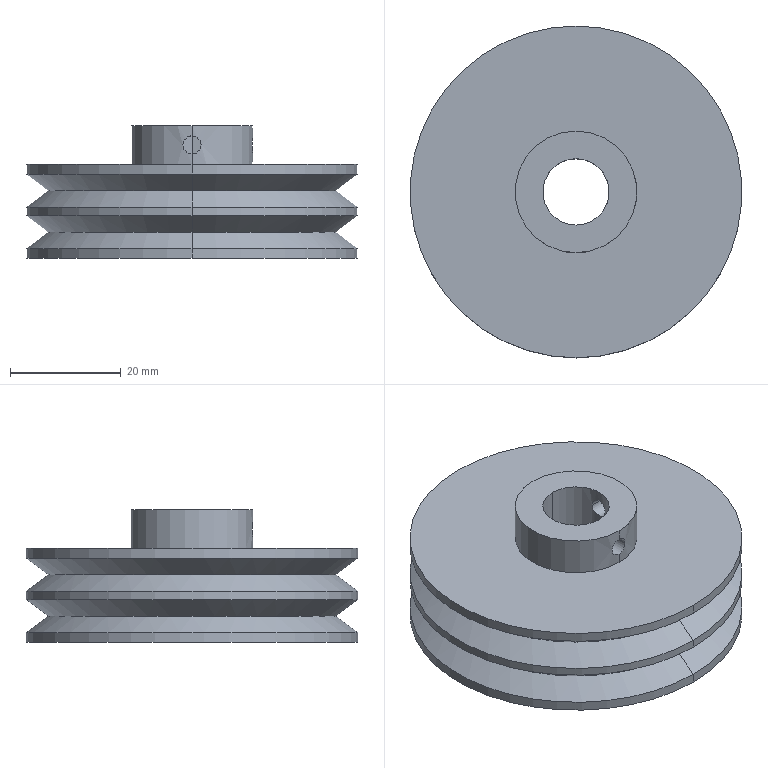Component | SolidWorks | MotorPulley-1 | 1 solid | 25 faces | box 60 x 60 x 24 mm | volume 43604 mm3 | cylinder 14 | cone 8 | plane 3 | commonest cylinder face diameters 60 x6 3.3 x4 22 x2 12 x2
build123d program:
from build123d import *


with BuildPart() as part:
    # Sketch1 → Revolve1 (revolve)
    with BuildSketch(Plane.XY, mode=Mode.PRIVATE) as revolve1_sk:
        Polygon((6, 50.885), (11, 50.885), (11, 43.885), (30, 43.885), (30, 42.135), (26, 39.135), (30, 36.135), (30, 34.635), (26, 31.635), (30, 28.635), (30, 26.885), (6, 26.885), align=None)
    revolve(revolve1_sk.sketch.rotate(Axis((0, 0, 0), (0, 1, 0)), 90), axis=Axis((0, 0, 0), (0, 1, 0)))

    # Sketch4 → M4 Tapped Hole4 (revolve, cut)
    with BuildSketch(Plane(origin=(0, 47.385, 0), x_dir=(0, 1, 0), z_dir=(1, 0, 0))):
        Polygon((0, 0), (0, 12.491), (1.65, 11.5), (1.65, 0), align=None)
    revolve(axis=Axis((0, 47.385, -6.35), (0, 0, 1)), mode=Mode.SUBTRACT)

    # Sketch6 → M4 Tapped Hole5 (revolve, cut)
    with BuildSketch(Plane.ZX.offset(47.385)):
        Polygon((0, 0), (0, 12.491), (1.65, 11.5), (1.65, 0), align=None)
    revolve(axis=Axis((-6.35, 47.385, 0), (1, 0, 0)), mode=Mode.SUBTRACT)


solid = part.part

# Placed as in the assembly
solid = solid.moved(Location((-160.944, 693.983, 228.904), (90, 0, 0)))
STEP:
#1=COLOUR_RGB('',0.7922,0.8196,0.9333);
#2=FILL_AREA_STYLE_COLOUR('',#1);
#3=FILL_AREA_STYLE('',(#2));
#4=SURFACE_STYLE_FILL_AREA(#3);
#5=SURFACE_SIDE_STYLE('',(#4));
#6=SURFACE_STYLE_USAGE(.BOTH.,#5);
#7=PRESENTATION_STYLE_ASSIGNMENT((#6));
#8=CARTESIAN_POINT('',(-5.908,27.257,10.878));
#9=VERTEX_POINT('',#8);
#10=CARTESIAN_POINT('',(-5.908,27.387,10.878));
#11=VERTEX_POINT('',#10);
#12=CARTESIAN_POINT('',(-5.908,27.257,10.878));
#13=CARTESIAN_POINT('',(-5.908,27.257,10.873));
#14=CARTESIAN_POINT('',(-5.908,27.258,10.869));
#15=CARTESIAN_POINT('',(-5.908,27.259,10.861));
#16=CARTESIAN_POINT('',(-5.908,27.261,10.857));
#17=CARTESIAN_POINT('',(-5.907,27.264,10.849));
#18=CARTESIAN_POINT('',(-5.907,27.266,10.845));
#19=CARTESIAN_POINT('',(-5.906,27.271,10.838));
#20=CARTESIAN_POINT('',(-5.906,27.273,10.835));
#21=CARTESIAN_POINT('',(-5.905,27.282,10.826));
#22=CARTESIAN_POINT('',(-5.904,27.289,10.821));
#23=CARTESIAN_POINT('',(-5.904,27.305,10.814));
#24=CARTESIAN_POINT('',(-5.903,27.314,10.813));
#25=CARTESIAN_POINT('',(-5.903,27.326,10.813));
#26=CARTESIAN_POINT('',(-5.903,27.331,10.813));
#27=CARTESIAN_POINT('',(-5.904,27.339,10.815));
#28=CARTESIAN_POINT('',(-5.904,27.343,10.816));
#29=CARTESIAN_POINT('',(-5.904,27.351,10.819));
#30=CARTESIAN_POINT('',(-5.905,27.355,10.821));
#31=CARTESIAN_POINT('',(-5.905,27.362,10.826));
#32=CARTESIAN_POINT('',(-5.905,27.365,10.829));
#33=CARTESIAN_POINT('',(-5.906,27.371,10.835));
#34=CARTESIAN_POINT('',(-5.906,27.374,10.838));
#35=CARTESIAN_POINT('',(-5.907,27.379,10.845));
#36=CARTESIAN_POINT('',(-5.907,27.381,10.849));
#37=CARTESIAN_POINT('',(-5.908,27.384,10.857));
#38=CARTESIAN_POINT('',(-5.908,27.385,10.861));
#39=CARTESIAN_POINT('',(-5.908,27.387,10.869));
#40=CARTESIAN_POINT('',(-5.908,27.387,10.873));
#41=CARTESIAN_POINT('',(-5.908,27.387,10.878));
#42=B_SPLINE_CURVE_WITH_KNOTS('',3,(#12,#13,#14,#15,#16,#17,#18,#19,#20,#21,#22,#23,#24,#25,#26,#27,#28,#29,#30,#31,#32,#33,#34,#35,#36,#37,#38,#39,#40,#41),.UNSPECIFIED.,.F.,.F.,(4,2,2,2,2,2,2,2,2,2,2,2,2,2,4),(0.,0.0003229,0.0006457,0.0009686,0.001291,0.001937,0.002583,0.002906,0.003229,0.003552,0.003874,0.004197,0.00452,0.004843,0.005166),.UNSPECIFIED.);
#43=EDGE_CURVE('',#9,#11,#42,.T.);
#44=ORIENTED_EDGE('',*,*,#43,.T.);
#45=CARTESIAN_POINT('',(-6.109,27.387,10.878));
#46=VERTEX_POINT('',#45);
#47=CARTESIAN_POINT('',(-6.336,27.387,10.878));
#48=DIRECTION('',(-1.,-0.,-0.));
#49=VECTOR('',#48,39.37);
#50=LINE('',#47,#49);
#51=EDGE_CURVE('',#11,#46,#50,.T.);
#52=ORIENTED_EDGE('',*,*,#51,.T.);
#53=CARTESIAN_POINT('',(-6.109,27.257,10.878));
#54=VERTEX_POINT('',#53);
#55=CARTESIAN_POINT('',(-6.109,27.387,10.878));
#56=CARTESIAN_POINT('',(-6.109,27.387,10.869));
#57=CARTESIAN_POINT('',(-6.109,27.385,10.86));
#58=CARTESIAN_POINT('',(-6.107,27.381,10.849));
#59=CARTESIAN_POINT('',(-6.107,27.379,10.845));
#60=CARTESIAN_POINT('',(-6.106,27.374,10.838));
#61=CARTESIAN_POINT('',(-6.105,27.371,10.835));
#62=CARTESIAN_POINT('',(-6.104,27.365,10.829));
#63=CARTESIAN_POINT('',(-6.103,27.362,10.826));
#64=CARTESIAN_POINT('',(-6.102,27.355,10.821));
#65=CARTESIAN_POINT('',(-6.102,27.351,10.819));
#66=CARTESIAN_POINT('',(-6.101,27.343,10.816));
#67=CARTESIAN_POINT('',(-6.101,27.339,10.815));
#68=CARTESIAN_POINT('',(-6.1,27.331,10.813));
#69=CARTESIAN_POINT('',(-6.1,27.326,10.813));
#70=CARTESIAN_POINT('',(-6.1,27.318,10.813));
#71=CARTESIAN_POINT('',(-6.1,27.314,10.813));
#72=CARTESIAN_POINT('',(-6.101,27.305,10.815));
#73=CARTESIAN_POINT('',(-6.101,27.301,10.816));
#74=CARTESIAN_POINT('',(-6.102,27.289,10.821));
#75=CARTESIAN_POINT('',(-6.103,27.282,10.826));
#76=CARTESIAN_POINT('',(-6.106,27.27,10.838));
#77=CARTESIAN_POINT('',(-6.107,27.265,10.845));
#78=CARTESIAN_POINT('',(-6.108,27.261,10.856));
#79=CARTESIAN_POINT('',(-6.109,27.259,10.861));
#80=CARTESIAN_POINT('',(-6.109,27.258,10.869));
#81=CARTESIAN_POINT('',(-6.109,27.257,10.873));
#82=CARTESIAN_POINT('',(-6.109,27.257,10.878));
#83=B_SPLINE_CURVE_WITH_KNOTS('',3,(#55,#56,#57,#58,#59,#60,#61,#62,#63,#64,#65,#66,#67,#68,#69,#70,#71,#72,#73,#74,#75,#76,#77,#78,#79,#80,#81,#82),.UNSPECIFIED.,.F.,.F.,(4,2,2,2,2,2,2,2,2,2,2,2,2,4),(0.005184,0.005831,0.006155,0.006479,0.006803,0.007127,0.007451,0.007775,0.008099,0.008423,0.00907,0.009718,0.01004,0.01037),.UNSPECIFIED.);
#84=EDGE_CURVE('',#46,#54,#83,.T.);
#85=ORIENTED_EDGE('',*,*,#84,.T.);
#86=CARTESIAN_POINT('',(-6.336,27.257,10.878));
#87=DIRECTION('',(-1.,-0.,-0.));
#88=VECTOR('',#87,39.37);
#89=LINE('',#86,#88);
#90=EDGE_CURVE('',#9,#54,#89,.T.);
#91=ORIENTED_EDGE('',*,*,#90,.F.);
#92=EDGE_LOOP('',(#44,#52,#85,#91));
#93=FACE_OUTER_BOUND('',#92,.T.);
#94=CARTESIAN_POINT('',(-6.336,27.322,10.878));
#95=DIRECTION('',(-1.,-0.,-0.));
#96=DIRECTION('',(0.,-1.,0.));
#97=AXIS2_PLACEMENT_3D('',#94,#95,#96);
#98=CYLINDRICAL_SURFACE('',#97,0.06496);
#99=ADVANCED_FACE('',(#93),#98,.F.);
#100=CARTESIAN_POINT('',(-6.336,26.889,10.813));
#101=VERTEX_POINT('',#100);
#102=CARTESIAN_POINT('',(-6.271,26.894,10.878));
#103=VERTEX_POINT('',#102);
#104=CARTESIAN_POINT('',(-6.336,26.889,10.813));
#105=CARTESIAN_POINT('',(-6.332,26.889,10.813));
#106=CARTESIAN_POINT('',(-6.328,26.889,10.813));
#107=CARTESIAN_POINT('',(-6.319,26.889,10.815));
#108=CARTESIAN_POINT('',(-6.315,26.89,10.816));
#109=CARTESIAN_POINT('',(-6.308,26.89,10.819));
#110=CARTESIAN_POINT('',(-6.304,26.89,10.821));
#111=CARTESIAN_POINT('',(-6.297,26.891,10.826));
#112=CARTESIAN_POINT('',(-6.293,26.891,10.829));
#113=CARTESIAN_POINT('',(-6.287,26.892,10.835));
#114=CARTESIAN_POINT('',(-6.285,26.892,10.838));
#115=CARTESIAN_POINT('',(-6.28,26.893,10.845));
#116=CARTESIAN_POINT('',(-6.278,26.893,10.849));
#117=CARTESIAN_POINT('',(-6.275,26.894,10.857));
#118=CARTESIAN_POINT('',(-6.273,26.894,10.861));
#119=CARTESIAN_POINT('',(-6.272,26.894,10.869));
#120=CARTESIAN_POINT('',(-6.271,26.894,10.873));
#121=CARTESIAN_POINT('',(-6.271,26.894,10.878));
#122=B_SPLINE_CURVE_WITH_KNOTS('',3,(#104,#105,#106,#107,#108,#109,#110,#111,#112,#113,#114,#115,#116,#117,#118,#119,#120,#121),.UNSPECIFIED.,.F.,.F.,(4,2,2,2,2,2,2,2,4),(0.002584,0.002906,0.003229,0.003552,0.003875,0.004198,0.00452,0.004843,0.005166),.UNSPECIFIED.);
#123=EDGE_CURVE('',#101,#103,#122,.T.);
#124=ORIENTED_EDGE('',*,*,#123,.T.);
#125=CARTESIAN_POINT('',(-6.271,27.095,10.878));
#126=VERTEX_POINT('',#125);
#127=CARTESIAN_POINT('',(-6.271,27.322,10.878));
#128=DIRECTION('',(-0.,1.,0.));
#129=VECTOR('',#128,39.37);
#130=LINE('',#127,#129);
#131=EDGE_CURVE('',#103,#126,#130,.T.);
#132=ORIENTED_EDGE('',*,*,#131,.T.);
#133=CARTESIAN_POINT('',(-6.336,27.086,10.813));
#134=VERTEX_POINT('',#133);
#135=CARTESIAN_POINT('',(-6.271,27.095,10.878));
#136=CARTESIAN_POINT('',(-6.271,27.095,10.869));
#137=CARTESIAN_POINT('',(-6.273,27.095,10.86));
#138=CARTESIAN_POINT('',(-6.278,27.093,10.849));
#139=CARTESIAN_POINT('',(-6.28,27.093,10.845));
#140=CARTESIAN_POINT('',(-6.285,27.092,10.838));
#141=CARTESIAN_POINT('',(-6.287,27.091,10.835));
#142=CARTESIAN_POINT('',(-6.293,27.09,10.829));
#143=CARTESIAN_POINT('',(-6.297,27.089,10.826));
#144=CARTESIAN_POINT('',(-6.304,27.088,10.821));
#145=CARTESIAN_POINT('',(-6.307,27.088,10.819));
#146=CARTESIAN_POINT('',(-6.315,27.087,10.816));
#147=CARTESIAN_POINT('',(-6.319,27.087,10.815));
#148=CARTESIAN_POINT('',(-6.328,27.086,10.813));
#149=CARTESIAN_POINT('',(-6.332,27.086,10.813));
#150=CARTESIAN_POINT('',(-6.336,27.086,10.813));
#151=B_SPLINE_CURVE_WITH_KNOTS('',3,(#135,#136,#137,#138,#139,#140,#141,#142,#143,#144,#145,#146,#147,#148,#149,#150),.UNSPECIFIED.,.F.,.F.,(4,2,2,2,2,2,2,4),(0.005184,0.005832,0.006155,0.006479,0.006803,0.007127,0.007451,0.007775),.UNSPECIFIED.);
#152=EDGE_CURVE('',#126,#134,#151,.T.);
#153=ORIENTED_EDGE('',*,*,#152,.T.);
#154=CARTESIAN_POINT('',(-6.401,27.095,10.878));
#155=VERTEX_POINT('',#154);
#156=CARTESIAN_POINT('',(-6.336,27.086,10.813));
#157=CARTESIAN_POINT('',(-6.341,27.086,10.813));
#158=CARTESIAN_POINT('',(-6.345,27.086,10.813));
#159=CARTESIAN_POINT('',(-6.353,27.087,10.815));
#160=CARTESIAN_POINT('',(-6.357,27.087,10.816));
#161=CARTESIAN_POINT('',(-6.369,27.088,10.821));
#162=CARTESIAN_POINT('',(-6.376,27.089,10.826));
#163=CARTESIAN_POINT('',(-6.388,27.092,10.838));
#164=CARTESIAN_POINT('',(-6.393,27.093,10.845));
#165=CARTESIAN_POINT('',(-6.398,27.094,10.856));
#166=CARTESIAN_POINT('',(-6.399,27.094,10.861));
#167=CARTESIAN_POINT('',(-6.401,27.095,10.869));
#168=CARTESIAN_POINT('',(-6.401,27.095,10.873));
#169=CARTESIAN_POINT('',(-6.401,27.095,10.878));
#170=B_SPLINE_CURVE_WITH_KNOTS('',3,(#156,#157,#158,#159,#160,#161,#162,#163,#164,#165,#166,#167,#168,#169),.UNSPECIFIED.,.F.,.F.,(4,2,2,2,2,2,4),(0.007775,0.008099,0.008423,0.009071,0.009718,0.01004,0.01037),.UNSPECIFIED.);
#171=EDGE_CURVE('',#134,#155,#170,.T.);
#172=ORIENTED_EDGE('',*,*,#171,.T.);
#173=CARTESIAN_POINT('',(-6.401,26.894,10.878));
#174=VERTEX_POINT('',#173);
#175=CARTESIAN_POINT('',(-6.401,27.322,10.878));
#176=DIRECTION('',(-0.,1.,0.));
#177=VECTOR('',#176,39.37);
#178=LINE('',#175,#177);
#179=EDGE_CURVE('',#174,#155,#178,.T.);
#180=ORIENTED_EDGE('',*,*,#179,.F.);
#181=CARTESIAN_POINT('',(-6.401,26.894,10.878));
#182=CARTESIAN_POINT('',(-6.401,26.894,10.873));
#183=CARTESIAN_POINT('',(-6.401,26.894,10.869));
#184=CARTESIAN_POINT('',(-6.399,26.894,10.861));
#185=CARTESIAN_POINT('',(-6.398,26.894,10.857));
#186=CARTESIAN_POINT('',(-6.395,26.893,10.849));
#187=CARTESIAN_POINT('',(-6.393,26.893,10.845));
#188=CARTESIAN_POINT('',(-6.388,26.892,10.838));
#189=CARTESIAN_POINT('',(-6.385,26.892,10.835));
#190=CARTESIAN_POINT('',(-6.376,26.891,10.826));
#191=CARTESIAN_POINT('',(-6.369,26.89,10.821));
#192=CARTESIAN_POINT('',(-6.353,26.889,10.814));
#193=CARTESIAN_POINT('',(-6.345,26.889,10.813));
#194=CARTESIAN_POINT('',(-6.336,26.889,10.813));
#195=B_SPLINE_CURVE_WITH_KNOTS('',3,(#181,#182,#183,#184,#185,#186,#187,#188,#189,#190,#191,#192,#193,#194),.UNSPECIFIED.,.F.,.F.,(4,2,2,2,2,2,4),(0.,0.0003229,0.0006459,0.0009688,0.001292,0.001938,0.002584),.UNSPECIFIED.);
#196=EDGE_CURVE('',#174,#101,#195,.T.);
#197=ORIENTED_EDGE('',*,*,#196,.T.);
#198=EDGE_LOOP('',(#124,#132,#153,#172,#180,#197));
#199=FACE_OUTER_BOUND('',#198,.T.);
#200=CARTESIAN_POINT('',(-6.336,27.322,10.878));
#201=DIRECTION('',(-0.,1.,0.));
#202=DIRECTION('',(-1.,0.,0.));
#203=AXIS2_PLACEMENT_3D('',#200,#201,#202);
#204=CYLINDRICAL_SURFACE('',#203,0.06496);
#205=ADVANCED_FACE('',(#199),#204,.F.);
#206=CARTESIAN_POINT('',(-6.336,28.503,10.139));
#207=VERTEX_POINT('',#206);
#208=CARTESIAN_POINT('',(-6.336,26.141,10.139));
#209=VERTEX_POINT('',#208);
#210=CARTESIAN_POINT('',(-6.336,27.322,10.139));
#211=DIRECTION('',(0.,0.,-1.));
#212=DIRECTION('',(0.,1.,0.));
#213=AXIS2_PLACEMENT_3D('',#210,#211,#212);
#214=CIRCLE('',#213,1.181);
#215=EDGE_CURVE('',#207,#209,#214,.T.);
#216=ORIENTED_EDGE('',*,*,#215,.T.);
#217=CARTESIAN_POINT('',(-6.336,26.141,10.07));
#218=VERTEX_POINT('',#217);
#219=CARTESIAN_POINT('',(-6.336,26.141,9.012));
#220=DIRECTION('',(0.,0.,-1.));
#221=VECTOR('',#220,39.37);
#222=LINE('',#219,#221);
#223=EDGE_CURVE('',#209,#218,#222,.T.);
#224=ORIENTED_EDGE('',*,*,#223,.T.);
#225=CARTESIAN_POINT('',(-6.336,28.503,10.07));
#226=VERTEX_POINT('',#225);
#227=CARTESIAN_POINT('',(-6.336,27.322,10.07));
#228=DIRECTION('',(0.,0.,-1.));
#229=DIRECTION('',(0.,1.,0.));
#230=AXIS2_PLACEMENT_3D('',#227,#228,#229);
#231=CIRCLE('',#230,1.181);
#232=EDGE_CURVE('',#226,#218,#231,.T.);
#233=ORIENTED_EDGE('',*,*,#232,.F.);
#234=CARTESIAN_POINT('',(-6.336,28.503,9.012));
#235=DIRECTION('',(0.,0.,-1.));
#236=VECTOR('',#235,39.37);
#237=LINE('',#234,#236);
#238=EDGE_CURVE('',#207,#226,#237,.T.);
#239=ORIENTED_EDGE('',*,*,#238,.F.);
#240=EDGE_LOOP('',(#216,#224,#233,#239));
#241=FACE_OUTER_BOUND('',#240,.T.);
#242=CARTESIAN_POINT('',(-6.336,27.322,9.012));
#243=DIRECTION('',(0.,0.,-1.));
#244=DIRECTION('',(0.,1.,0.));
#245=AXIS2_PLACEMENT_3D('',#242,#243,#244);
#246=CYLINDRICAL_SURFACE('',#245,1.181);
#247=ADVANCED_FACE('',(#241),#246,.T.);
#248=CARTESIAN_POINT('',(-6.336,28.346,10.257));
#249=VERTEX_POINT('',#248);
#250=CARTESIAN_POINT('',(-6.336,26.299,10.257));
#251=VERTEX_POINT('',#250);
#252=CARTESIAN_POINT('',(-6.336,27.322,10.257));
#253=DIRECTION('',(0.,0.,-1.));
#254=DIRECTION('',(0.,1.,0.));
#255=AXIS2_PLACEMENT_3D('',#252,#253,#254);
#256=CIRCLE('',#255,1.024);
#257=EDGE_CURVE('',#249,#251,#256,.T.);
#258=ORIENTED_EDGE('',*,*,#257,.T.);
#259=CARTESIAN_POINT('',(-6.336,26.141,10.139));
#260=DIRECTION('',(0.,-0.8,-0.6));
#261=VECTOR('',#260,39.37);
#262=LINE('',#259,#261);
#263=EDGE_CURVE('',#251,#209,#262,.T.);
#264=ORIENTED_EDGE('',*,*,#263,.T.);
#265=ORIENTED_EDGE('',*,*,#215,.F.);
#266=CARTESIAN_POINT('',(-6.336,28.503,10.139));
#267=DIRECTION('',(-0.,0.8,-0.6));
#268=VECTOR('',#267,39.37);
#269=LINE('',#266,#268);
#270=EDGE_CURVE('',#249,#207,#269,.T.);
#271=ORIENTED_EDGE('',*,*,#270,.F.);
#272=EDGE_LOOP('',(#258,#264,#265,#271));
#273=FACE_OUTER_BOUND('',#272,.T.);
#274=CARTESIAN_POINT('',(-6.336,27.322,10.139));
#275=DIRECTION('',(0.,0.,-1.));
#276=DIRECTION('',(0.,1.,0.));
#277=AXIS2_PLACEMENT_3D('',#274,#275,#276);
#278=CONICAL_SURFACE('',#277,1.181,0.9273);
#279=ADVANCED_FACE('',(#273),#278,.T.);
#280=ORIENTED_EDGE('',*,*,#257,.F.);
#281=CARTESIAN_POINT('',(-6.336,28.503,10.376));
#282=VERTEX_POINT('',#281);
#283=CARTESIAN_POINT('',(-6.336,28.346,10.257));
#284=DIRECTION('',(0.,0.8,0.6));
#285=VECTOR('',#284,39.37);
#286=LINE('',#283,#285);
#287=EDGE_CURVE('',#249,#282,#286,.T.);
#288=ORIENTED_EDGE('',*,*,#287,.T.);
#289=CARTESIAN_POINT('',(-6.336,26.141,10.376));
#290=VERTEX_POINT('',#289);
#291=CARTESIAN_POINT('',(-6.336,27.322,10.376));
#292=DIRECTION('',(0.,0.,-1.));
#293=DIRECTION('',(0.,1.,0.));
#294=AXIS2_PLACEMENT_3D('',#291,#292,#293);
#295=CIRCLE('',#294,1.181);
#296=EDGE_CURVE('',#282,#290,#295,.T.);
#297=ORIENTED_EDGE('',*,*,#296,.T.);
#298=CARTESIAN_POINT('',(-6.336,26.299,10.257));
#299=DIRECTION('',(0.,-0.8,0.6));
#300=VECTOR('',#299,39.37);
#301=LINE('',#298,#300);
#302=EDGE_CURVE('',#251,#290,#301,.T.);
#303=ORIENTED_EDGE('',*,*,#302,.F.);
#304=EDGE_LOOP('',(#280,#288,#297,#303));
#305=FACE_OUTER_BOUND('',#304,.T.);
#306=CARTESIAN_POINT('',(-6.336,27.322,10.257));
#307=DIRECTION('',(-0.,-0.,1.));
#308=DIRECTION('',(0.,-1.,0.));
#309=AXIS2_PLACEMENT_3D('',#306,#307,#308);
#310=CONICAL_SURFACE('',#309,1.024,0.9273);
#311=ADVANCED_FACE('',(#305),#310,.T.);
#312=CARTESIAN_POINT('',(-6.336,28.503,10.435));
#313=VERTEX_POINT('',#312);
#314=CARTESIAN_POINT('',(-6.336,26.141,10.435));
#315=VERTEX_POINT('',#314);
#316=CARTESIAN_POINT('',(-6.336,27.322,10.435));
#317=DIRECTION('',(0.,0.,-1.));
#318=DIRECTION('',(0.,1.,0.));
#319=AXIS2_PLACEMENT_3D('',#316,#317,#318);
#320=CIRCLE('',#319,1.181);
#321=EDGE_CURVE('',#313,#315,#320,.T.);
#322=ORIENTED_EDGE('',*,*,#321,.T.);
#323=CARTESIAN_POINT('',(-6.336,26.141,9.012));
#324=DIRECTION('',(0.,0.,-1.));
#325=VECTOR('',#324,39.37);
#326=LINE('',#323,#325);
#327=EDGE_CURVE('',#315,#290,#326,.T.);
#328=ORIENTED_EDGE('',*,*,#327,.T.);
#329=ORIENTED_EDGE('',*,*,#296,.F.);
#330=CARTESIAN_POINT('',(-6.336,28.503,9.012));
#331=DIRECTION('',(0.,0.,-1.));
#332=VECTOR('',#331,39.37);
#333=LINE('',#330,#332);
#334=EDGE_CURVE('',#313,#282,#333,.T.);
#335=ORIENTED_EDGE('',*,*,#334,.F.);
#336=EDGE_LOOP('',(#322,#328,#329,#335));
#337=FACE_OUTER_BOUND('',#336,.T.);
#338=CARTESIAN_POINT('',(-6.336,27.322,9.012));
#339=DIRECTION('',(0.,0.,-1.));
#340=DIRECTION('',(0.,1.,0.));
#341=AXIS2_PLACEMENT_3D('',#338,#339,#340);
#342=CYLINDRICAL_SURFACE('',#341,1.181);
#343=ADVANCED_FACE('',(#337),#342,.T.);
#344=CARTESIAN_POINT('',(-6.336,28.346,10.553));
#345=VERTEX_POINT('',#344);
#346=CARTESIAN_POINT('',(-6.336,26.299,10.553));
#347=VERTEX_POINT('',#346);
#348=CARTESIAN_POINT('',(-6.336,27.322,10.553));
#349=DIRECTION('',(0.,0.,-1.));
#350=DIRECTION('',(0.,1.,0.));
#351=AXIS2_PLACEMENT_3D('',#348,#349,#350);
#352=CIRCLE('',#351,1.024);
#353=EDGE_CURVE('',#345,#347,#352,.T.);
#354=ORIENTED_EDGE('',*,*,#353,.T.);
#355=CARTESIAN_POINT('',(-6.336,26.141,10.435));
#356=DIRECTION('',(0.,-0.8,-0.6));
#357=VECTOR('',#356,39.37);
#358=LINE('',#355,#357);
#359=EDGE_CURVE('',#347,#315,#358,.T.);
#360=ORIENTED_EDGE('',*,*,#359,.T.);
#361=ORIENTED_EDGE('',*,*,#321,.F.);
#362=CARTESIAN_POINT('',(-6.336,28.503,10.435));
#363=DIRECTION('',(-0.,0.8,-0.6));
#364=VECTOR('',#363,39.37);
#365=LINE('',#362,#364);
#366=EDGE_CURVE('',#345,#313,#365,.T.);
#367=ORIENTED_EDGE('',*,*,#366,.F.);
#368=EDGE_LOOP('',(#354,#360,#361,#367));
#369=FACE_OUTER_BOUND('',#368,.T.);
#370=CARTESIAN_POINT('',(-6.336,27.322,10.435));
#371=DIRECTION('',(0.,0.,-1.));
#372=DIRECTION('',(0.,1.,0.));
#373=AXIS2_PLACEMENT_3D('',#370,#371,#372);
#374=CONICAL_SURFACE('',#373,1.181,0.9273);
#375=ADVANCED_FACE('',(#369),#374,.T.);
#376=ORIENTED_EDGE('',*,*,#353,.F.);
#377=CARTESIAN_POINT('',(-6.336,28.503,10.671));
#378=VERTEX_POINT('',#377);
#379=CARTESIAN_POINT('',(-6.336,28.346,10.553));
#380=DIRECTION('',(0.,0.8,0.6));
#381=VECTOR('',#380,39.37);
#382=LINE('',#379,#381);
#383=EDGE_CURVE('',#345,#378,#382,.T.);
#384=ORIENTED_EDGE('',*,*,#383,.T.);
#385=CARTESIAN_POINT('',(-6.336,26.141,10.671));
#386=VERTEX_POINT('',#385);
#387=CARTESIAN_POINT('',(-6.336,27.322,10.671));
#388=DIRECTION('',(0.,0.,-1.));
#389=DIRECTION('',(0.,1.,0.));
#390=AXIS2_PLACEMENT_3D('',#387,#388,#389);
#391=CIRCLE('',#390,1.181);
#392=EDGE_CURVE('',#378,#386,#391,.T.);
#393=ORIENTED_EDGE('',*,*,#392,.T.);
#394=CARTESIAN_POINT('',(-6.336,26.299,10.553));
#395=DIRECTION('',(0.,-0.8,0.6));
#396=VECTOR('',#395,39.37);
#397=LINE('',#394,#396);
#398=EDGE_CURVE('',#347,#386,#397,.T.);
#399=ORIENTED_EDGE('',*,*,#398,.F.);
#400=EDGE_LOOP('',(#376,#384,#393,#399));
#401=FACE_OUTER_BOUND('',#400,.T.);
#402=CARTESIAN_POINT('',(-6.336,27.322,10.553));
#403=DIRECTION('',(-0.,-0.,1.));
#404=DIRECTION('',(0.,-1.,0.));
#405=AXIS2_PLACEMENT_3D('',#402,#403,#404);
#406=CONICAL_SURFACE('',#405,1.024,0.9273);
#407=ADVANCED_FACE('',(#401),#406,.T.);
#408=CARTESIAN_POINT('',(-6.336,28.503,10.74));
#409=VERTEX_POINT('',#408);
#410=CARTESIAN_POINT('',(-6.336,26.141,10.74));
#411=VERTEX_POINT('',#410);
#412=CARTESIAN_POINT('',(-6.336,27.322,10.74));
#413=DIRECTION('',(0.,0.,-1.));
#414=DIRECTION('',(0.,1.,0.));
#415=AXIS2_PLACEMENT_3D('',#412,#413,#414);
#416=CIRCLE('',#415,1.181);
#417=EDGE_CURVE('',#409,#411,#416,.T.);
#418=ORIENTED_EDGE('',*,*,#417,.T.);
#419=CARTESIAN_POINT('',(-6.336,26.141,9.012));
#420=DIRECTION('',(0.,0.,-1.));
#421=VECTOR('',#420,39.37);
#422=LINE('',#419,#421);
#423=EDGE_CURVE('',#411,#386,#422,.T.);
#424=ORIENTED_EDGE('',*,*,#423,.T.);
#425=ORIENTED_EDGE('',*,*,#392,.F.);
#426=CARTESIAN_POINT('',(-6.336,28.503,9.012));
#427=DIRECTION('',(0.,0.,-1.));
#428=VECTOR('',#427,39.37);
#429=LINE('',#426,#428);
#430=EDGE_CURVE('',#409,#378,#429,.T.);
#431=ORIENTED_EDGE('',*,*,#430,.F.);
#432=EDGE_LOOP('',(#418,#424,#425,#431));
#433=FACE_OUTER_BOUND('',#432,.T.);
#434=CARTESIAN_POINT('',(-6.336,27.322,9.012));
#435=DIRECTION('',(0.,0.,-1.));
#436=DIRECTION('',(0.,1.,0.));
#437=AXIS2_PLACEMENT_3D('',#434,#435,#436);
#438=CYLINDRICAL_SURFACE('',#437,1.181);
#439=ADVANCED_FACE('',(#433),#438,.T.);
#440=ORIENTED_EDGE('',*,*,#43,.F.);
#441=CARTESIAN_POINT('',(-5.908,27.387,10.878));
#442=CARTESIAN_POINT('',(-5.908,27.387,10.886));
#443=CARTESIAN_POINT('',(-5.908,27.385,10.895));
#444=CARTESIAN_POINT('',(-5.907,27.379,10.91));
#445=CARTESIAN_POINT('',(-5.906,27.374,10.917));
#446=CARTESIAN_POINT('',(-5.905,27.365,10.926));
#447=CARTESIAN_POINT('',(-5.905,27.362,10.929));
#448=CARTESIAN_POINT('',(-5.905,27.355,10.934));
#449=CARTESIAN_POINT('',(-5.904,27.351,10.936));
#450=CARTESIAN_POINT('',(-5.904,27.343,10.939));
#451=CARTESIAN_POINT('',(-5.904,27.339,10.94));
#452=CARTESIAN_POINT('',(-5.903,27.331,10.942));
#453=CARTESIAN_POINT('',(-5.903,27.327,10.942));
#454=CARTESIAN_POINT('',(-5.903,27.318,10.942));
#455=CARTESIAN_POINT('',(-5.903,27.314,10.942));
#456=CARTESIAN_POINT('',(-5.904,27.305,10.94));
#457=CARTESIAN_POINT('',(-5.904,27.301,10.939));
#458=CARTESIAN_POINT('',(-5.904,27.293,10.936));
#459=CARTESIAN_POINT('',(-5.904,27.29,10.934));
#460=CARTESIAN_POINT('',(-5.905,27.283,10.929));
#461=CARTESIAN_POINT('',(-5.905,27.279,10.926));
#462=CARTESIAN_POINT('',(-5.906,27.27,10.917));
#463=CARTESIAN_POINT('',(-5.907,27.265,10.91));
#464=CARTESIAN_POINT('',(-5.908,27.259,10.895));
#465=CARTESIAN_POINT('',(-5.908,27.257,10.886));
#466=CARTESIAN_POINT('',(-5.908,27.257,10.878));
#467=B_SPLINE_CURVE_WITH_KNOTS('',3,(#441,#442,#443,#444,#445,#446,#447,#448,#449,#450,#451,#452,#453,#454,#455,#456,#457,#458,#459,#460,#461,#462,#463,#464,#465,#466),.UNSPECIFIED.,.F.,.F.,(4,2,2,2,2,2,2,2,2,2,2,2,4),(0.005166,0.005812,0.006457,0.00678,0.007103,0.007425,0.007748,0.008071,0.008394,0.008717,0.009039,0.009685,0.01033),.UNSPECIFIED.);
#468=EDGE_CURVE('',#11,#9,#467,.T.);
#469=ORIENTED_EDGE('',*,*,#468,.F.);
#470=EDGE_LOOP('',(#440,#469));
#471=FACE_BOUND('',#470,.T.);
#472=CARTESIAN_POINT('',(-6.336,27.755,11.015));
#473=VERTEX_POINT('',#472);
#474=CARTESIAN_POINT('',(-6.336,26.889,11.015));
#475=VERTEX_POINT('',#474);
#476=CARTESIAN_POINT('',(-6.336,27.322,11.015));
#477=DIRECTION('',(0.,0.,-1.));
#478=DIRECTION('',(0.,1.,0.));
#479=AXIS2_PLACEMENT_3D('',#476,#477,#478);
#480=CIRCLE('',#479,0.4331);
#481=EDGE_CURVE('',#473,#475,#480,.T.);
#482=ORIENTED_EDGE('',*,*,#481,.T.);
#483=CARTESIAN_POINT('',(-6.336,26.889,10.942));
#484=VERTEX_POINT('',#483);
#485=CARTESIAN_POINT('',(-6.336,26.889,9.012));
#486=DIRECTION('',(0.,0.,-1.));
#487=VECTOR('',#486,39.37);
#488=LINE('',#485,#487);
#489=EDGE_CURVE('',#475,#484,#488,.T.);
#490=ORIENTED_EDGE('',*,*,#489,.T.);
#491=CARTESIAN_POINT('',(-6.271,26.894,10.878));
#492=CARTESIAN_POINT('',(-6.271,26.894,10.886));
#493=CARTESIAN_POINT('',(-6.273,26.894,10.895));
#494=CARTESIAN_POINT('',(-6.28,26.893,10.91));
#495=CARTESIAN_POINT('',(-6.284,26.892,10.917));
#496=CARTESIAN_POINT('',(-6.293,26.891,10.926));
#497=CARTESIAN_POINT('',(-6.297,26.891,10.929));
#498=CARTESIAN_POINT('',(-6.304,26.89,10.934));
#499=CARTESIAN_POINT('',(-6.308,26.89,10.936));
#500=CARTESIAN_POINT('',(-6.319,26.889,10.941));
#501=CARTESIAN_POINT('',(-6.328,26.889,10.942));
#502=CARTESIAN_POINT('',(-6.336,26.889,10.942));
#503=B_SPLINE_CURVE_WITH_KNOTS('',3,(#491,#492,#493,#494,#495,#496,#497,#498,#499,#500,#501,#502),.UNSPECIFIED.,.F.,.F.,(4,2,2,2,2,4),(0.005166,0.005812,0.006458,0.006781,0.007103,0.007749),.UNSPECIFIED.);
#504=EDGE_CURVE('',#103,#484,#503,.T.);
#505=ORIENTED_EDGE('',*,*,#504,.F.);
#506=ORIENTED_EDGE('',*,*,#123,.F.);
#507=CARTESIAN_POINT('',(-6.336,26.889,10.74));
#508=VERTEX_POINT('',#507);
#509=CARTESIAN_POINT('',(-6.336,26.889,9.012));
#510=DIRECTION('',(0.,0.,-1.));
#511=VECTOR('',#510,39.37);
#512=LINE('',#509,#511);
#513=EDGE_CURVE('',#101,#508,#512,.T.);
#514=ORIENTED_EDGE('',*,*,#513,.T.);
#515=CARTESIAN_POINT('',(-6.336,27.755,10.74));
#516=VERTEX_POINT('',#515);
#517=CARTESIAN_POINT('',(-6.336,27.322,10.74));
#518=DIRECTION('',(0.,0.,-1.));
#519=DIRECTION('',(0.,1.,0.));
#520=AXIS2_PLACEMENT_3D('',#517,#518,#519);
#521=CIRCLE('',#520,0.4331);
#522=EDGE_CURVE('',#516,#508,#521,.T.);
#523=ORIENTED_EDGE('',*,*,#522,.F.);
#524=CARTESIAN_POINT('',(-6.336,27.755,9.012));
#525=DIRECTION('',(0.,0.,-1.));
#526=VECTOR('',#525,39.37);
#527=LINE('',#524,#526);
#528=EDGE_CURVE('',#473,#516,#527,.T.);
#529=ORIENTED_EDGE('',*,*,#528,.F.);
#530=EDGE_LOOP('',(#482,#490,#505,#506,#514,#523,#529));
#531=FACE_OUTER_BOUND('',#530,.T.);
#532=CARTESIAN_POINT('',(-6.336,27.322,9.012));
#533=DIRECTION('',(0.,0.,-1.));
#534=DIRECTION('',(0.,1.,0.));
#535=AXIS2_PLACEMENT_3D('',#532,#533,#534);
#536=CYLINDRICAL_SURFACE('',#535,0.4331);
#537=ADVANCED_FACE('',(#471,#531),#536,.T.);
#538=CARTESIAN_POINT('',(-6.336,27.086,11.015));
#539=VERTEX_POINT('',#538);
#540=CARTESIAN_POINT('',(-6.336,27.558,11.015));
#541=VERTEX_POINT('',#540);
#542=CARTESIAN_POINT('',(-6.336,27.322,11.015));
#543=DIRECTION('',(0.,0.,-1.));
#544=DIRECTION('',(0.,1.,0.));
#545=AXIS2_PLACEMENT_3D('',#542,#543,#544);
#546=CIRCLE('',#545,0.2362);
#547=EDGE_CURVE('',#539,#541,#546,.T.);
#548=ORIENTED_EDGE('',*,*,#547,.F.);
#549=CARTESIAN_POINT('',(-6.336,27.086,10.942));
#550=VERTEX_POINT('',#549);
#551=CARTESIAN_POINT('',(-6.336,27.086,9.012));
#552=DIRECTION('',(0.,0.,-1.));
#553=VECTOR('',#552,39.37);
#554=LINE('',#551,#553);
#555=EDGE_CURVE('',#539,#550,#554,.T.);
#556=ORIENTED_EDGE('',*,*,#555,.T.);
#557=CARTESIAN_POINT('',(-6.401,27.095,10.878));
#558=CARTESIAN_POINT('',(-6.401,27.095,10.882));
#559=CARTESIAN_POINT('',(-6.401,27.095,10.886));
#560=CARTESIAN_POINT('',(-6.399,27.094,10.894));
#561=CARTESIAN_POINT('',(-6.398,27.094,10.899));
#562=CARTESIAN_POINT('',(-6.395,27.093,10.906));
#563=CARTESIAN_POINT('',(-6.393,27.093,10.91));
#564=CARTESIAN_POINT('',(-6.388,27.092,10.917));
#565=CARTESIAN_POINT('',(-6.385,27.091,10.92));
#566=CARTESIAN_POINT('',(-6.376,27.089,10.929));
#567=CARTESIAN_POINT('',(-6.369,27.088,10.934));
#568=CARTESIAN_POINT('',(-6.353,27.086,10.941));
#569=CARTESIAN_POINT('',(-6.345,27.086,10.942));
#570=CARTESIAN_POINT('',(-6.336,27.086,10.942));
#571=B_SPLINE_CURVE_WITH_KNOTS('',3,(#557,#558,#559,#560,#561,#562,#563,#564,#565,#566,#567,#568,#569,#570),.UNSPECIFIED.,.F.,.F.,(4,2,2,2,2,2,4),(0.,0.0003241,0.0006481,0.0009722,0.001296,0.001944,0.002593),.UNSPECIFIED.);
#572=EDGE_CURVE('',#155,#550,#571,.T.);
#573=ORIENTED_EDGE('',*,*,#572,.F.);
#574=ORIENTED_EDGE('',*,*,#171,.F.);
#575=CARTESIAN_POINT('',(-6.336,27.086,10.07));
#576=VERTEX_POINT('',#575);
#577=CARTESIAN_POINT('',(-6.336,27.086,9.012));
#578=DIRECTION('',(0.,0.,-1.));
#579=VECTOR('',#578,39.37);
#580=LINE('',#577,#579);
#581=EDGE_CURVE('',#134,#576,#580,.T.);
#582=ORIENTED_EDGE('',*,*,#581,.T.);
#583=CARTESIAN_POINT('',(-6.336,27.558,10.07));
#584=VERTEX_POINT('',#583);
#585=CARTESIAN_POINT('',(-6.336,27.322,10.07));
#586=DIRECTION('',(0.,0.,-1.));
#587=DIRECTION('',(0.,1.,0.));
#588=AXIS2_PLACEMENT_3D('',#585,#586,#587);
#589=CIRCLE('',#588,0.2362);
#590=EDGE_CURVE('',#576,#584,#589,.T.);
#591=ORIENTED_EDGE('',*,*,#590,.T.);
#592=CARTESIAN_POINT('',(-6.336,27.558,9.012));
#593=DIRECTION('',(0.,0.,-1.));
#594=VECTOR('',#593,39.37);
#595=LINE('',#592,#594);
#596=EDGE_CURVE('',#541,#584,#595,.T.);
#597=ORIENTED_EDGE('',*,*,#596,.F.);
#598=EDGE_LOOP('',(#548,#556,#573,#574,#582,#591,#597));
#599=FACE_OUTER_BOUND('',#598,.T.);
#600=CARTESIAN_POINT('',(-6.336,27.322,9.012));
#601=DIRECTION('',(0.,0.,-1.));
#602=DIRECTION('',(0.,1.,0.));
#603=AXIS2_PLACEMENT_3D('',#600,#601,#602);
#604=CYLINDRICAL_SURFACE('',#603,0.2362);
#605=ADVANCED_FACE('',(#599),#604,.F.);
#606=ORIENTED_EDGE('',*,*,#555,.F.);
#607=CARTESIAN_POINT('',(-6.336,27.322,11.015));
#608=DIRECTION('',(0.,0.,-1.));
#609=DIRECTION('',(0.,1.,0.));
#610=AXIS2_PLACEMENT_3D('',#607,#608,#609);
#611=CIRCLE('',#610,0.2362);
#612=EDGE_CURVE('',#541,#539,#611,.T.);
#613=ORIENTED_EDGE('',*,*,#612,.F.);
#614=ORIENTED_EDGE('',*,*,#596,.T.);
#615=CARTESIAN_POINT('',(-6.336,27.322,10.07));
#616=DIRECTION('',(0.,0.,-1.));
#617=DIRECTION('',(0.,1.,0.));
#618=AXIS2_PLACEMENT_3D('',#615,#616,#617);
#619=CIRCLE('',#618,0.2362);
#620=EDGE_CURVE('',#584,#576,#619,.T.);
#621=ORIENTED_EDGE('',*,*,#620,.T.);
#622=ORIENTED_EDGE('',*,*,#581,.F.);
#623=ORIENTED_EDGE('',*,*,#152,.F.);
#624=CARTESIAN_POINT('',(-6.336,27.086,10.942));
#625=CARTESIAN_POINT('',(-6.332,27.086,10.942));
#626=CARTESIAN_POINT('',(-6.328,27.086,10.942));
#627=CARTESIAN_POINT('',(-6.319,27.087,10.94));
#628=CARTESIAN_POINT('',(-6.315,27.087,10.939));
#629=CARTESIAN_POINT('',(-6.304,27.088,10.934));
#630=CARTESIAN_POINT('',(-6.296,27.089,10.929));
#631=CARTESIAN_POINT('',(-6.287,27.091,10.92));
#632=CARTESIAN_POINT('',(-6.285,27.092,10.917));
#633=CARTESIAN_POINT('',(-6.28,27.093,10.91));
#634=CARTESIAN_POINT('',(-6.278,27.093,10.906));
#635=CARTESIAN_POINT('',(-6.275,27.094,10.898));
#636=CARTESIAN_POINT('',(-6.274,27.094,10.894));
#637=CARTESIAN_POINT('',(-6.272,27.095,10.886));
#638=CARTESIAN_POINT('',(-6.271,27.095,10.882));
#639=CARTESIAN_POINT('',(-6.271,27.095,10.878));
#640=B_SPLINE_CURVE_WITH_KNOTS('',3,(#624,#625,#626,#627,#628,#629,#630,#631,#632,#633,#634,#635,#636,#637,#638,#639),.UNSPECIFIED.,.F.,.F.,(4,2,2,2,2,2,2,4),(0.002593,0.002916,0.00324,0.003888,0.004212,0.004536,0.00486,0.005184),.UNSPECIFIED.);
#641=EDGE_CURVE('',#550,#126,#640,.T.);
#642=ORIENTED_EDGE('',*,*,#641,.F.);
#643=EDGE_LOOP('',(#606,#613,#614,#621,#622,#623,#642));
#644=FACE_OUTER_BOUND('',#643,.T.);
#645=CARTESIAN_POINT('',(-6.109,27.257,10.878));
#646=CARTESIAN_POINT('',(-6.109,27.257,10.882));
#647=CARTESIAN_POINT('',(-6.109,27.258,10.886));
#648=CARTESIAN_POINT('',(-6.109,27.259,10.894));
#649=CARTESIAN_POINT('',(-6.108,27.261,10.899));
#650=CARTESIAN_POINT('',(-6.107,27.264,10.906));
#651=CARTESIAN_POINT('',(-6.107,27.266,10.91));
#652=CARTESIAN_POINT('',(-6.106,27.271,10.917));
#653=CARTESIAN_POINT('',(-6.105,27.273,10.92));
#654=CARTESIAN_POINT('',(-6.103,27.282,10.929));
#655=CARTESIAN_POINT('',(-6.102,27.289,10.934));
#656=CARTESIAN_POINT('',(-6.101,27.305,10.941));
#657=CARTESIAN_POINT('',(-6.1,27.314,10.942));
#658=CARTESIAN_POINT('',(-6.1,27.326,10.942));
#659=CARTESIAN_POINT('',(-6.1,27.331,10.942));
#660=CARTESIAN_POINT('',(-6.101,27.339,10.94));
#661=CARTESIAN_POINT('',(-6.101,27.343,10.939));
#662=CARTESIAN_POINT('',(-6.102,27.355,10.934));
#663=CARTESIAN_POINT('',(-6.103,27.362,10.929));
#664=CARTESIAN_POINT('',(-6.105,27.371,10.92));
#665=CARTESIAN_POINT('',(-6.106,27.374,10.917));
#666=CARTESIAN_POINT('',(-6.107,27.379,10.91));
#667=CARTESIAN_POINT('',(-6.107,27.381,10.906));
#668=CARTESIAN_POINT('',(-6.108,27.384,10.899));
#669=CARTESIAN_POINT('',(-6.109,27.385,10.894));
#670=CARTESIAN_POINT('',(-6.109,27.387,10.886));
#671=CARTESIAN_POINT('',(-6.109,27.387,10.882));
#672=CARTESIAN_POINT('',(-6.109,27.387,10.878));
#673=B_SPLINE_CURVE_WITH_KNOTS('',3,(#645,#646,#647,#648,#649,#650,#651,#652,#653,#654,#655,#656,#657,#658,#659,#660,#661,#662,#663,#664,#665,#666,#667,#668,#669,#670,#671,#672),.UNSPECIFIED.,.F.,.F.,(4,2,2,2,2,2,2,2,2,2,2,2,2,4),(0.,0.000324,0.000648,0.0009719,0.001296,0.001944,0.002592,0.002916,0.00324,0.003888,0.004212,0.004536,0.00486,0.005184),.UNSPECIFIED.);
#674=EDGE_CURVE('',#54,#46,#673,.T.);
#675=ORIENTED_EDGE('',*,*,#674,.F.);
#676=ORIENTED_EDGE('',*,*,#84,.F.);
#677=EDGE_LOOP('',(#675,#676));
#678=FACE_BOUND('',#677,.T.);
#679=CARTESIAN_POINT('',(-6.336,27.322,9.012));
#680=DIRECTION('',(0.,0.,-1.));
#681=DIRECTION('',(0.,1.,0.));
#682=AXIS2_PLACEMENT_3D('',#679,#680,#681);
#683=CYLINDRICAL_SURFACE('',#682,0.2362);
#684=ADVANCED_FACE('',(#644,#678),#683,.F.);
#685=ORIENTED_EDGE('',*,*,#612,.T.);
#686=ORIENTED_EDGE('',*,*,#547,.T.);
#687=EDGE_LOOP('',(#685,#686));
#688=FACE_BOUND('',#687,.T.);
#689=ORIENTED_EDGE('',*,*,#481,.F.);
#690=CARTESIAN_POINT('',(-6.336,27.322,11.015));
#691=DIRECTION('',(0.,0.,-1.));
#692=DIRECTION('',(0.,1.,0.));
#693=AXIS2_PLACEMENT_3D('',#690,#691,#692);
#694=CIRCLE('',#693,0.4331);
#695=EDGE_CURVE('',#475,#473,#694,.T.);
#696=ORIENTED_EDGE('',*,*,#695,.F.);
#697=EDGE_LOOP('',(#689,#696));
#698=FACE_OUTER_BOUND('',#697,.T.);
#699=CARTESIAN_POINT('',(-6.1,27.322,11.015));
#700=DIRECTION('',(-0.,-0.,1.));
#701=DIRECTION('',(0.,-1.,-0.));
#702=AXIS2_PLACEMENT_3D('',#699,#700,#701);
#703=PLANE('',#702);
#704=ADVANCED_FACE('',(#688,#698),#703,.T.);
#705=ORIENTED_EDGE('',*,*,#489,.F.);
#706=ORIENTED_EDGE('',*,*,#695,.T.);
#707=ORIENTED_EDGE('',*,*,#528,.T.);
#708=CARTESIAN_POINT('',(-6.336,27.322,10.74));
#709=DIRECTION('',(0.,0.,-1.));
#710=DIRECTION('',(0.,1.,0.));
#711=AXIS2_PLACEMENT_3D('',#708,#709,#710);
#712=CIRCLE('',#711,0.4331);
#713=EDGE_CURVE('',#508,#516,#712,.T.);
#714=ORIENTED_EDGE('',*,*,#713,.F.);
#715=ORIENTED_EDGE('',*,*,#513,.F.);
#716=ORIENTED_EDGE('',*,*,#196,.F.);
#717=CARTESIAN_POINT('',(-6.336,26.889,10.942));
#718=CARTESIAN_POINT('',(-6.341,26.889,10.942));
#719=CARTESIAN_POINT('',(-6.345,26.889,10.942));
#720=CARTESIAN_POINT('',(-6.353,26.889,10.94));
#721=CARTESIAN_POINT('',(-6.357,26.89,10.939));
#722=CARTESIAN_POINT('',(-6.365,26.89,10.936));
#723=CARTESIAN_POINT('',(-6.369,26.89,10.934));
#724=CARTESIAN_POINT('',(-6.376,26.891,10.929));
#725=CARTESIAN_POINT('',(-6.379,26.891,10.926));
#726=CARTESIAN_POINT('',(-6.388,26.892,10.917));
#727=CARTESIAN_POINT('',(-6.393,26.893,10.91));
#728=CARTESIAN_POINT('',(-6.4,26.894,10.895));
#729=CARTESIAN_POINT('',(-6.401,26.894,10.886));
#730=CARTESIAN_POINT('',(-6.401,26.894,10.878));
#731=B_SPLINE_CURVE_WITH_KNOTS('',3,(#717,#718,#719,#720,#721,#722,#723,#724,#725,#726,#727,#728,#729,#730),.UNSPECIFIED.,.F.,.F.,(4,2,2,2,2,2,4),(0.007749,0.008072,0.008395,0.008717,0.00904,0.009685,0.01033),.UNSPECIFIED.);
#732=EDGE_CURVE('',#484,#174,#731,.T.);
#733=ORIENTED_EDGE('',*,*,#732,.F.);
#734=EDGE_LOOP('',(#705,#706,#707,#714,#715,#716,#733));
#735=FACE_OUTER_BOUND('',#734,.T.);
#736=CARTESIAN_POINT('',(-6.336,27.322,9.012));
#737=DIRECTION('',(0.,0.,-1.));
#738=DIRECTION('',(0.,1.,0.));
#739=AXIS2_PLACEMENT_3D('',#736,#737,#738);
#740=CYLINDRICAL_SURFACE('',#739,0.4331);
#741=ADVANCED_FACE('',(#735),#740,.T.);
#742=ORIENTED_EDGE('',*,*,#522,.T.);
#743=ORIENTED_EDGE('',*,*,#713,.T.);
#744=EDGE_LOOP('',(#742,#743));
#745=FACE_BOUND('',#744,.T.);
#746=ORIENTED_EDGE('',*,*,#417,.F.);
#747=CARTESIAN_POINT('',(-6.336,27.322,10.74));
#748=DIRECTION('',(0.,0.,-1.));
#749=DIRECTION('',(0.,1.,0.));
#750=AXIS2_PLACEMENT_3D('',#747,#748,#749);
#751=CIRCLE('',#750,1.181);
#752=EDGE_CURVE('',#411,#409,#751,.T.);
#753=ORIENTED_EDGE('',*,*,#752,.F.);
#754=EDGE_LOOP('',(#746,#753));
#755=FACE_OUTER_BOUND('',#754,.T.);
#756=CARTESIAN_POINT('',(-5.903,27.322,10.74));
#757=DIRECTION('',(-0.,-0.,1.));
#758=DIRECTION('',(0.,-1.,-0.));
#759=AXIS2_PLACEMENT_3D('',#756,#757,#758);
#760=PLANE('',#759);
#761=ADVANCED_FACE('',(#745,#755),#760,.T.);
#762=ORIENTED_EDGE('',*,*,#423,.F.);
#763=ORIENTED_EDGE('',*,*,#752,.T.);
#764=ORIENTED_EDGE('',*,*,#430,.T.);
#765=CARTESIAN_POINT('',(-6.336,27.322,10.671));
#766=DIRECTION('',(0.,0.,-1.));
#767=DIRECTION('',(0.,1.,0.));
#768=AXIS2_PLACEMENT_3D('',#765,#766,#767);
#769=CIRCLE('',#768,1.181);
#770=EDGE_CURVE('',#386,#378,#769,.T.);
#771=ORIENTED_EDGE('',*,*,#770,.F.);
#772=EDGE_LOOP('',(#762,#763,#764,#771));
#773=FACE_OUTER_BOUND('',#772,.T.);
#774=CARTESIAN_POINT('',(-6.336,27.322,9.012));
#775=DIRECTION('',(0.,0.,-1.));
#776=DIRECTION('',(0.,1.,0.));
#777=AXIS2_PLACEMENT_3D('',#774,#775,#776);
#778=CYLINDRICAL_SURFACE('',#777,1.181);
#779=ADVANCED_FACE('',(#773),#778,.T.);
#780=ORIENTED_EDGE('',*,*,#383,.F.);
#781=CARTESIAN_POINT('',(-6.336,27.322,10.553));
#782=DIRECTION('',(0.,0.,-1.));
#783=DIRECTION('',(0.,1.,0.));
#784=AXIS2_PLACEMENT_3D('',#781,#782,#783);
#785=CIRCLE('',#784,1.024);
#786=EDGE_CURVE('',#347,#345,#785,.T.);
#787=ORIENTED_EDGE('',*,*,#786,.F.);
#788=ORIENTED_EDGE('',*,*,#398,.T.);
#789=ORIENTED_EDGE('',*,*,#770,.T.);
#790=EDGE_LOOP('',(#780,#787,#788,#789));
#791=FACE_OUTER_BOUND('',#790,.T.);
#792=CARTESIAN_POINT('',(-6.336,27.322,10.553));
#793=DIRECTION('',(-0.,-0.,1.));
#794=DIRECTION('',(0.,-1.,0.));
#795=AXIS2_PLACEMENT_3D('',#792,#793,#794);
#796=CONICAL_SURFACE('',#795,1.024,0.9273);
#797=ADVANCED_FACE('',(#791),#796,.T.);
#798=ORIENTED_EDGE('',*,*,#359,.F.);
#799=ORIENTED_EDGE('',*,*,#786,.T.);
#800=ORIENTED_EDGE('',*,*,#366,.T.);
#801=CARTESIAN_POINT('',(-6.336,27.322,10.435));
#802=DIRECTION('',(0.,0.,-1.));
#803=DIRECTION('',(0.,1.,0.));
#804=AXIS2_PLACEMENT_3D('',#801,#802,#803);
#805=CIRCLE('',#804,1.181);
#806=EDGE_CURVE('',#315,#313,#805,.T.);
#807=ORIENTED_EDGE('',*,*,#806,.F.);
#808=EDGE_LOOP('',(#798,#799,#800,#807));
#809=FACE_OUTER_BOUND('',#808,.T.);
#810=CARTESIAN_POINT('',(-6.336,27.322,10.435));
#811=DIRECTION('',(0.,0.,-1.));
#812=DIRECTION('',(0.,1.,0.));
#813=AXIS2_PLACEMENT_3D('',#810,#811,#812);
#814=CONICAL_SURFACE('',#813,1.181,0.9273);
#815=ADVANCED_FACE('',(#809),#814,.T.);
#816=ORIENTED_EDGE('',*,*,#327,.F.);
#817=ORIENTED_EDGE('',*,*,#806,.T.);
#818=ORIENTED_EDGE('',*,*,#334,.T.);
#819=CARTESIAN_POINT('',(-6.336,27.322,10.376));
#820=DIRECTION('',(0.,0.,-1.));
#821=DIRECTION('',(0.,1.,0.));
#822=AXIS2_PLACEMENT_3D('',#819,#820,#821);
#823=CIRCLE('',#822,1.181);
#824=EDGE_CURVE('',#290,#282,#823,.T.);
#825=ORIENTED_EDGE('',*,*,#824,.F.);
#826=EDGE_LOOP('',(#816,#817,#818,#825));
#827=FACE_OUTER_BOUND('',#826,.T.);
#828=CARTESIAN_POINT('',(-6.336,27.322,9.012));
#829=DIRECTION('',(0.,0.,-1.));
#830=DIRECTION('',(0.,1.,0.));
#831=AXIS2_PLACEMENT_3D('',#828,#829,#830);
#832=CYLINDRICAL_SURFACE('',#831,1.181);
#833=ADVANCED_FACE('',(#827),#832,.T.);
#834=ORIENTED_EDGE('',*,*,#287,.F.);
#835=CARTESIAN_POINT('',(-6.336,27.322,10.257));
#836=DIRECTION('',(0.,0.,-1.));
#837=DIRECTION('',(0.,1.,0.));
#838=AXIS2_PLACEMENT_3D('',#835,#836,#837);
#839=CIRCLE('',#838,1.024);
#840=EDGE_CURVE('',#251,#249,#839,.T.);
#841=ORIENTED_EDGE('',*,*,#840,.F.);
#842=ORIENTED_EDGE('',*,*,#302,.T.);
#843=ORIENTED_EDGE('',*,*,#824,.T.);
#844=EDGE_LOOP('',(#834,#841,#842,#843));
#845=FACE_OUTER_BOUND('',#844,.T.);
#846=CARTESIAN_POINT('',(-6.336,27.322,10.257));
#847=DIRECTION('',(-0.,-0.,1.));
#848=DIRECTION('',(0.,-1.,0.));
#849=AXIS2_PLACEMENT_3D('',#846,#847,#848);
#850=CONICAL_SURFACE('',#849,1.024,0.9273);
#851=ADVANCED_FACE('',(#845),#850,.T.);
#852=ORIENTED_EDGE('',*,*,#263,.F.);
#853=ORIENTED_EDGE('',*,*,#840,.T.);
#854=ORIENTED_EDGE('',*,*,#270,.T.);
#855=CARTESIAN_POINT('',(-6.336,27.322,10.139));
#856=DIRECTION('',(0.,0.,-1.));
#857=DIRECTION('',(0.,1.,0.));
#858=AXIS2_PLACEMENT_3D('',#855,#856,#857);
#859=CIRCLE('',#858,1.181);
#860=EDGE_CURVE('',#209,#207,#859,.T.);
#861=ORIENTED_EDGE('',*,*,#860,.F.);
#862=EDGE_LOOP('',(#852,#853,#854,#861));
#863=FACE_OUTER_BOUND('',#862,.T.);
#864=CARTESIAN_POINT('',(-6.336,27.322,10.139));
#865=DIRECTION('',(0.,0.,-1.));
#866=DIRECTION('',(0.,1.,0.));
#867=AXIS2_PLACEMENT_3D('',#864,#865,#866);
#868=CONICAL_SURFACE('',#867,1.181,0.9273);
#869=ADVANCED_FACE('',(#863),#868,.T.);
#870=ORIENTED_EDGE('',*,*,#223,.F.);
#871=ORIENTED_EDGE('',*,*,#860,.T.);
#872=ORIENTED_EDGE('',*,*,#238,.T.);
#873=CARTESIAN_POINT('',(-6.336,27.322,10.07));
#874=DIRECTION('',(0.,0.,-1.));
#875=DIRECTION('',(0.,1.,0.));
#876=AXIS2_PLACEMENT_3D('',#873,#874,#875);
#877=CIRCLE('',#876,1.181);
#878=EDGE_CURVE('',#218,#226,#877,.T.);
#879=ORIENTED_EDGE('',*,*,#878,.F.);
#880=EDGE_LOOP('',(#870,#871,#872,#879));
#881=FACE_OUTER_BOUND('',#880,.T.);
#882=CARTESIAN_POINT('',(-6.336,27.322,9.012));
#883=DIRECTION('',(0.,0.,-1.));
#884=DIRECTION('',(0.,1.,0.));
#885=AXIS2_PLACEMENT_3D('',#882,#883,#884);
#886=CYLINDRICAL_SURFACE('',#885,1.181);
#887=ADVANCED_FACE('',(#881),#886,.T.);
#888=ORIENTED_EDGE('',*,*,#232,.T.);
#889=ORIENTED_EDGE('',*,*,#878,.T.);
#890=EDGE_LOOP('',(#888,#889));
#891=FACE_OUTER_BOUND('',#890,.T.);
#892=ORIENTED_EDGE('',*,*,#620,.F.);
#893=ORIENTED_EDGE('',*,*,#590,.F.);
#894=EDGE_LOOP('',(#892,#893));
#895=FACE_BOUND('',#894,.T.);
#896=CARTESIAN_POINT('',(-5.155,27.322,10.07));
#897=DIRECTION('',(0.,0.,-1.));
#898=DIRECTION('',(-0.,1.,0.));
#899=AXIS2_PLACEMENT_3D('',#896,#897,#898);
#900=PLANE('',#899);
#901=ADVANCED_FACE('',(#891,#895),#900,.T.);
#902=ORIENTED_EDGE('',*,*,#131,.F.);
#903=ORIENTED_EDGE('',*,*,#504,.T.);
#904=ORIENTED_EDGE('',*,*,#732,.T.);
#905=ORIENTED_EDGE('',*,*,#179,.T.);
#906=ORIENTED_EDGE('',*,*,#572,.T.);
#907=ORIENTED_EDGE('',*,*,#641,.T.);
#908=EDGE_LOOP('',(#902,#903,#904,#905,#906,#907));
#909=FACE_OUTER_BOUND('',#908,.T.);
#910=CARTESIAN_POINT('',(-6.336,27.322,10.878));
#911=DIRECTION('',(-0.,1.,0.));
#912=DIRECTION('',(-1.,0.,0.));
#913=AXIS2_PLACEMENT_3D('',#910,#911,#912);
#914=CYLINDRICAL_SURFACE('',#913,0.06496);
#915=ADVANCED_FACE('',(#909),#914,.F.);
#916=ORIENTED_EDGE('',*,*,#51,.F.);
#917=ORIENTED_EDGE('',*,*,#468,.T.);
#918=ORIENTED_EDGE('',*,*,#90,.T.);
#919=ORIENTED_EDGE('',*,*,#674,.T.);
#920=EDGE_LOOP('',(#916,#917,#918,#919));
#921=FACE_OUTER_BOUND('',#920,.T.);
#922=CARTESIAN_POINT('',(-6.336,27.322,10.878));
#923=DIRECTION('',(-1.,-0.,-0.));
#924=DIRECTION('',(0.,-1.,0.));
#925=AXIS2_PLACEMENT_3D('',#922,#923,#924);
#926=CYLINDRICAL_SURFACE('',#925,0.06496);
#927=ADVANCED_FACE('',(#921),#926,.F.);
#928=CLOSED_SHELL('',(#99,#205,#247,#279,#311,#343,#375,#407,#439,#537,#605,#684,#704,#741,#761,#779,#797,#815,#833,#851,#869,#887,#901,#915,#927));
#929=MANIFOLD_SOLID_BREP('',#928);
#930=STYLED_ITEM('',(#7),#929);
#931=PRESENTATION_LAYER_ASSIGNMENT('','',(#930));
#932=CARTESIAN_POINT('',(0.,0.,0.));
#933=DIRECTION('',(0.,0.,1.));
#934=DIRECTION('',(1.,0.,0.));
#935=AXIS2_PLACEMENT_3D('',#932,#933,#934);
#936=(LENGTH_UNIT()NAMED_UNIT(*)SI_UNIT($,.METRE.));
#937=LENGTH_MEASURE_WITH_UNIT(LENGTH_MEASURE(0.0254),#936);
#938=DIMENSIONAL_EXPONENTS(1.,0.,0.,0.,0.,0.,0.);
#939=(CONVERSION_BASED_UNIT('',#937)LENGTH_UNIT()NAMED_UNIT(#938));
#940=UNCERTAINTY_MEASURE_WITH_UNIT(LENGTH_MEASURE(0.00001),#939,'','');
#941=(NAMED_UNIT(*)PLANE_ANGLE_UNIT()SI_UNIT($,.RADIAN.));
#942=(NAMED_UNIT(*)SI_UNIT($,.STERADIAN.)SOLID_ANGLE_UNIT());
#943=(GEOMETRIC_REPRESENTATION_CONTEXT(3)GLOBAL_UNCERTAINTY_ASSIGNED_CONTEXT((#940))GLOBAL_UNIT_ASSIGNED_CONTEXT((#939,#941,#942))REPRESENTATION_CONTEXT('',''));
#944=ADVANCED_BREP_SHAPE_REPRESENTATION('',(#929,#935),#943);
#945=(LENGTH_UNIT()NAMED_UNIT(*)SI_UNIT($,.METRE.));
#946=LENGTH_MEASURE_WITH_UNIT(LENGTH_MEASURE(0.0254),#945);
#947=DIMENSIONAL_EXPONENTS(1.,0.,0.,0.,0.,0.,0.);
#948=(CONVERSION_BASED_UNIT('',#946)LENGTH_UNIT()NAMED_UNIT(#947));
#949=UNCERTAINTY_MEASURE_WITH_UNIT(LENGTH_MEASURE(0.00001),#948,'','');
#950=(NAMED_UNIT(*)PLANE_ANGLE_UNIT()SI_UNIT($,.RADIAN.));
#951=(NAMED_UNIT(*)SI_UNIT($,.STERADIAN.)SOLID_ANGLE_UNIT());
#952=(GEOMETRIC_REPRESENTATION_CONTEXT(3)GLOBAL_UNCERTAINTY_ASSIGNED_CONTEXT((#949))GLOBAL_UNIT_ASSIGNED_CONTEXT((#948,#950,#951))REPRESENTATION_CONTEXT('',''));
#953=MECHANICAL_DESIGN_GEOMETRIC_PRESENTATION_REPRESENTATION('',(#930),#952);